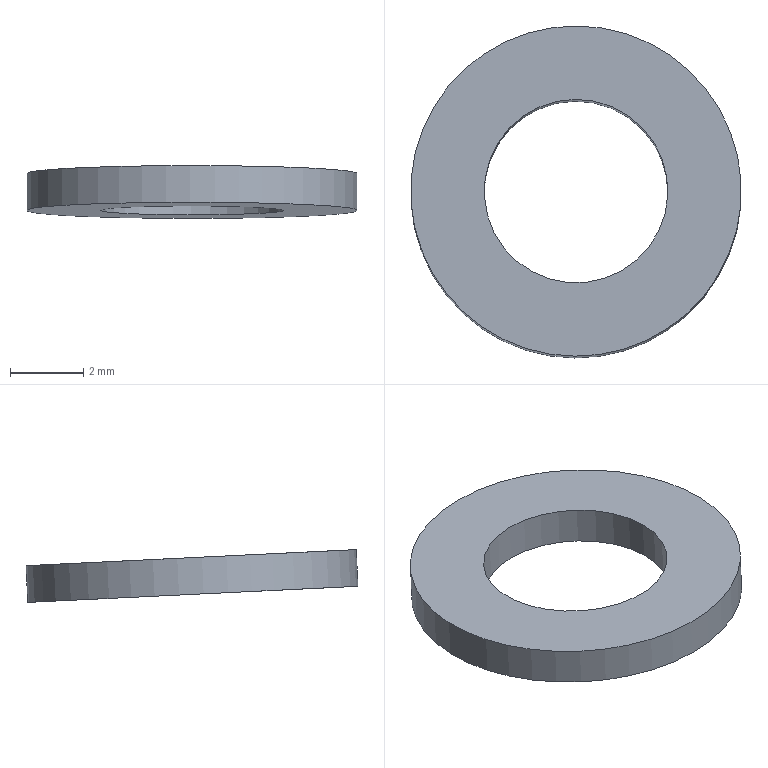Component | NX | CCJ-023 | 1 solid | 4 faces | box 9 x 9.04 x 1.44 mm | volume 44 mm3 | plane 2 | cylinder 2 | commonest cylinder face diameters 9 x1 5 x1
STEP:
#1=CARTESIAN_POINT('',(0.,0.,0.));
#2=DIRECTION('',(0.,0.,1.));
#3=DIRECTION('',(1.,0.,0.));
#4=AXIS2_PLACEMENT_3D('',#1,#2,#3);
#5=CARTESIAN_POINT('',(14.204,431.357,209.068));
#6=VERTEX_POINT('',#5);
#7=CARTESIAN_POINT('',(10.,429.754,209.146));
#8=DIRECTION('',(0.,-0.04861,-0.9988));
#9=DIRECTION('',(0.9342,0.3563,-0.01734));
#10=AXIS2_PLACEMENT_3D('',#7,#8,#9);
#11=CIRCLE('',#10,4.5);
#12=CARTESIAN_POINT('',(10.,429.754,209.146));
#13=DIRECTION('',(0.,0.04861,0.9988));
#14=DIRECTION('',(-0.9342,-0.3563,0.01734));
#15=AXIS2_PLACEMENT_3D('',#12,#13,#14);
#16=PLANE('',#15);
#17=CARTESIAN_POINT('',(-4.5,0.));
#18=CARTESIAN_POINT('',(-4.5,7.794));
#19=CARTESIAN_POINT('',(2.25,3.897));
#20=CARTESIAN_POINT('',(9.,-0.));
#21=CARTESIAN_POINT('',(2.25,-3.897));
#22=CARTESIAN_POINT('',(-4.5,-7.794));
#23=CARTESIAN_POINT('',(-4.5,0.));
#24=(BOUNDED_CURVE()B_SPLINE_CURVE(2,(#17,#18,#19,#20,#21,#22,#23),.UNSPECIFIED.,.T.,.F.)B_SPLINE_CURVE_WITH_KNOTS((1,2,2,2,2,1),(-2.094,0.,2.094,4.189,6.283,8.378),.UNSPECIFIED.)CURVE()GEOMETRIC_REPRESENTATION_ITEM()RATIONAL_B_SPLINE_CURVE((1.,0.5,1.,0.5,1.,0.5,1.))REPRESENTATION_ITEM(''));
#25=(GEOMETRIC_REPRESENTATION_CONTEXT(2)PARAMETRIC_REPRESENTATION_CONTEXT()REPRESENTATION_CONTEXT('',''));
#26=DEFINITIONAL_REPRESENTATION('',(#24),#25);
#27=PCURVE('',#16,#26);
#28=CARTESIAN_POINT('',(10.,429.754,209.146));
#29=DIRECTION('',(0.,-0.04861,-0.9988));
#30=DIRECTION('',(0.9342,0.3563,-0.01734));
#31=AXIS2_PLACEMENT_3D('',#28,#29,#30);
#32=CYLINDRICAL_SURFACE('',#31,4.5);
#33=CARTESIAN_POINT('',(0.,0.));
#34=DIRECTION('',(1.,0.));
#35=VECTOR('',#34,1.);
#36=LINE('',#33,#35);
#37=(GEOMETRIC_REPRESENTATION_CONTEXT(2)PARAMETRIC_REPRESENTATION_CONTEXT()REPRESENTATION_CONTEXT('',''));
#38=DEFINITIONAL_REPRESENTATION('',(#36),#37);
#39=PCURVE('',#32,#38);
#40=SURFACE_CURVE('',#11,(#27,#39),.PCURVE_S1.);
#41=EDGE_CURVE('',#6,#6,#40,.T.);
#42=ORIENTED_EDGE('',*,*,#41,.F.);
#43=EDGE_LOOP('',(#42));
#44=FACE_BOUND('',#43,.T.);
#45=CARTESIAN_POINT('',(12.336,430.645,209.103));
#46=VERTEX_POINT('',#45);
#47=CARTESIAN_POINT('',(10.,429.754,209.146));
#48=DIRECTION('',(0.,-0.04861,-0.9988));
#49=DIRECTION('',(0.9342,0.3563,-0.01734));
#50=AXIS2_PLACEMENT_3D('',#47,#48,#49);
#51=CIRCLE('',#50,2.5);
#52=CARTESIAN_POINT('',(-2.5,-0.));
#53=CARTESIAN_POINT('',(-2.5,4.33));
#54=CARTESIAN_POINT('',(1.25,2.165));
#55=CARTESIAN_POINT('',(5.,0.));
#56=CARTESIAN_POINT('',(1.25,-2.165));
#57=CARTESIAN_POINT('',(-2.5,-4.33));
#58=CARTESIAN_POINT('',(-2.5,-0.));
#59=(BOUNDED_CURVE()B_SPLINE_CURVE(2,(#52,#53,#54,#55,#56,#57,#58),.UNSPECIFIED.,.T.,.F.)B_SPLINE_CURVE_WITH_KNOTS((1,2,2,2,2,1),(-2.094,0.,2.094,4.189,6.283,8.378),.UNSPECIFIED.)CURVE()GEOMETRIC_REPRESENTATION_ITEM()RATIONAL_B_SPLINE_CURVE((1.,0.5,1.,0.5,1.,0.5,1.))REPRESENTATION_ITEM(''));
#60=(GEOMETRIC_REPRESENTATION_CONTEXT(2)PARAMETRIC_REPRESENTATION_CONTEXT()REPRESENTATION_CONTEXT('',''));
#61=DEFINITIONAL_REPRESENTATION('',(#59),#60);
#62=PCURVE('',#16,#61);
#63=CARTESIAN_POINT('',(10.,429.754,209.146));
#64=DIRECTION('',(0.,-0.04861,-0.9988));
#65=DIRECTION('',(0.9342,0.3563,-0.01734));
#66=AXIS2_PLACEMENT_3D('',#63,#64,#65);
#67=CYLINDRICAL_SURFACE('',#66,2.5);
#68=CARTESIAN_POINT('',(0.,-0.));
#69=DIRECTION('',(1.,0.));
#70=VECTOR('',#69,1.);
#71=LINE('',#68,#70);
#72=(GEOMETRIC_REPRESENTATION_CONTEXT(2)PARAMETRIC_REPRESENTATION_CONTEXT()REPRESENTATION_CONTEXT('',''));
#73=DEFINITIONAL_REPRESENTATION('',(#71),#72);
#74=PCURVE('',#67,#73);
#75=SURFACE_CURVE('',#51,(#62,#74),.PCURVE_S1.);
#76=EDGE_CURVE('',#46,#46,#75,.T.);
#77=ORIENTED_EDGE('',*,*,#76,.T.);
#78=EDGE_LOOP('',(#77));
#79=FACE_BOUND('',#78,.T.);
#80=ADVANCED_FACE('',(#44,#79),#16,.T.);
#81=CARTESIAN_POINT('',(14.204,431.309,208.069));
#82=VERTEX_POINT('',#81);
#83=CARTESIAN_POINT('',(10.,429.705,208.147));
#84=DIRECTION('',(0.,-0.04861,-0.9988));
#85=DIRECTION('',(0.9342,0.3563,-0.01734));
#86=AXIS2_PLACEMENT_3D('',#83,#84,#85);
#87=CIRCLE('',#86,4.5);
#88=CARTESIAN_POINT('',(10.,429.705,208.147));
#89=DIRECTION('',(0.,0.04861,0.9988));
#90=DIRECTION('',(-0.9342,-0.3563,0.01734));
#91=AXIS2_PLACEMENT_3D('',#88,#89,#90);
#92=PLANE('',#91);
#93=CARTESIAN_POINT('',(-4.5,0.));
#94=CARTESIAN_POINT('',(-4.5,7.794));
#95=CARTESIAN_POINT('',(2.25,3.897));
#96=CARTESIAN_POINT('',(9.,-0.));
#97=CARTESIAN_POINT('',(2.25,-3.897));
#98=CARTESIAN_POINT('',(-4.5,-7.794));
#99=CARTESIAN_POINT('',(-4.5,0.));
#100=(BOUNDED_CURVE()B_SPLINE_CURVE(2,(#93,#94,#95,#96,#97,#98,#99),.UNSPECIFIED.,.T.,.F.)B_SPLINE_CURVE_WITH_KNOTS((1,2,2,2,2,1),(-2.094,0.,2.094,4.189,6.283,8.378),.UNSPECIFIED.)CURVE()GEOMETRIC_REPRESENTATION_ITEM()RATIONAL_B_SPLINE_CURVE((1.,0.5,1.,0.5,1.,0.5,1.))REPRESENTATION_ITEM(''));
#101=(GEOMETRIC_REPRESENTATION_CONTEXT(2)PARAMETRIC_REPRESENTATION_CONTEXT()REPRESENTATION_CONTEXT('',''));
#102=DEFINITIONAL_REPRESENTATION('',(#100),#101);
#103=PCURVE('',#92,#102);
#104=CARTESIAN_POINT('',(0.,1.));
#105=DIRECTION('',(1.,0.));
#106=VECTOR('',#105,1.);
#107=LINE('',#104,#106);
#108=(GEOMETRIC_REPRESENTATION_CONTEXT(2)PARAMETRIC_REPRESENTATION_CONTEXT()REPRESENTATION_CONTEXT('',''));
#109=DEFINITIONAL_REPRESENTATION('',(#107),#108);
#110=PCURVE('',#32,#109);
#111=SURFACE_CURVE('',#87,(#103,#110),.PCURVE_S1.);
#112=EDGE_CURVE('',#82,#82,#111,.T.);
#113=ORIENTED_EDGE('',*,*,#112,.T.);
#114=EDGE_LOOP('',(#113));
#115=FACE_BOUND('',#114,.T.);
#116=CARTESIAN_POINT('',(12.336,430.596,208.104));
#117=VERTEX_POINT('',#116);
#118=CARTESIAN_POINT('',(10.,429.705,208.147));
#119=DIRECTION('',(0.,-0.04861,-0.9988));
#120=DIRECTION('',(0.9342,0.3563,-0.01734));
#121=AXIS2_PLACEMENT_3D('',#118,#119,#120);
#122=CIRCLE('',#121,2.5);
#123=CARTESIAN_POINT('',(-2.5,-0.));
#124=CARTESIAN_POINT('',(-2.5,4.33));
#125=CARTESIAN_POINT('',(1.25,2.165));
#126=CARTESIAN_POINT('',(5.,0.));
#127=CARTESIAN_POINT('',(1.25,-2.165));
#128=CARTESIAN_POINT('',(-2.5,-4.33));
#129=CARTESIAN_POINT('',(-2.5,-0.));
#130=(BOUNDED_CURVE()B_SPLINE_CURVE(2,(#123,#124,#125,#126,#127,#128,#129),.UNSPECIFIED.,.T.,.F.)B_SPLINE_CURVE_WITH_KNOTS((1,2,2,2,2,1),(-2.094,0.,2.094,4.189,6.283,8.378),.UNSPECIFIED.)CURVE()GEOMETRIC_REPRESENTATION_ITEM()RATIONAL_B_SPLINE_CURVE((1.,0.5,1.,0.5,1.,0.5,1.))REPRESENTATION_ITEM(''));
#131=(GEOMETRIC_REPRESENTATION_CONTEXT(2)PARAMETRIC_REPRESENTATION_CONTEXT()REPRESENTATION_CONTEXT('',''));
#132=DEFINITIONAL_REPRESENTATION('',(#130),#131);
#133=PCURVE('',#92,#132);
#134=CARTESIAN_POINT('',(0.,1.));
#135=DIRECTION('',(1.,0.));
#136=VECTOR('',#135,1.);
#137=LINE('',#134,#136);
#138=(GEOMETRIC_REPRESENTATION_CONTEXT(2)PARAMETRIC_REPRESENTATION_CONTEXT()REPRESENTATION_CONTEXT('',''));
#139=DEFINITIONAL_REPRESENTATION('',(#137),#138);
#140=PCURVE('',#67,#139);
#141=SURFACE_CURVE('',#122,(#133,#140),.PCURVE_S1.);
#142=EDGE_CURVE('',#117,#117,#141,.T.);
#143=ORIENTED_EDGE('',*,*,#142,.F.);
#144=EDGE_LOOP('',(#143));
#145=FACE_BOUND('',#144,.T.);
#146=ADVANCED_FACE('',(#115,#145),#92,.F.);
#147=ORIENTED_EDGE('',*,*,#41,.T.);
#148=CARTESIAN_POINT('',(14.204,431.357,209.068));
#149=CARTESIAN_POINT('',(14.204,431.309,208.069));
#150=B_SPLINE_CURVE_WITH_KNOTS('',1,(#148,#149),.UNSPECIFIED.,.F.,.F.,(2,2),(0.,1.),.PIECEWISE_BEZIER_KNOTS.);
#151=CARTESIAN_POINT('',(6.283,0.));
#152=DIRECTION('',(0.,1.));
#153=VECTOR('',#152,1.);
#154=LINE('',#151,#153);
#155=(GEOMETRIC_REPRESENTATION_CONTEXT(2)PARAMETRIC_REPRESENTATION_CONTEXT()REPRESENTATION_CONTEXT('',''));
#156=DEFINITIONAL_REPRESENTATION('',(#154),#155);
#157=PCURVE('',#32,#156);
#158=CARTESIAN_POINT('',(0.,0.));
#159=DIRECTION('',(0.,1.));
#160=VECTOR('',#159,1.);
#161=LINE('',#158,#160);
#162=(GEOMETRIC_REPRESENTATION_CONTEXT(2)PARAMETRIC_REPRESENTATION_CONTEXT()REPRESENTATION_CONTEXT('',''));
#163=DEFINITIONAL_REPRESENTATION('',(#161),#162);
#164=PCURVE('',#32,#163);
#165=SEAM_CURVE('',#150,(#157,#164),.PCURVE_S1.);
#166=EDGE_CURVE('',#6,#82,#165,.T.);
#167=ORIENTED_EDGE('',*,*,#166,.T.);
#168=ORIENTED_EDGE('',*,*,#112,.F.);
#169=ORIENTED_EDGE('',*,*,#166,.F.);
#170=EDGE_LOOP('',(#147,#167,#168,#169));
#171=FACE_BOUND('',#170,.T.);
#172=ADVANCED_FACE('',(#171),#32,.T.);
#173=ORIENTED_EDGE('',*,*,#76,.T.);
#174=CARTESIAN_POINT('',(12.336,430.645,209.103));
#175=CARTESIAN_POINT('',(12.336,430.596,208.104));
#176=B_SPLINE_CURVE_WITH_KNOTS('',1,(#174,#175),.UNSPECIFIED.,.F.,.F.,(2,2),(-0.,1.),.PIECEWISE_BEZIER_KNOTS.);
#177=CARTESIAN_POINT('',(6.283,0.));
#178=DIRECTION('',(0.,1.));
#179=VECTOR('',#178,1.);
#180=LINE('',#177,#179);
#181=(GEOMETRIC_REPRESENTATION_CONTEXT(2)PARAMETRIC_REPRESENTATION_CONTEXT()REPRESENTATION_CONTEXT('',''));
#182=DEFINITIONAL_REPRESENTATION('',(#180),#181);
#183=PCURVE('',#67,#182);
#184=CARTESIAN_POINT('',(0.,0.));
#185=DIRECTION('',(0.,1.));
#186=VECTOR('',#185,1.);
#187=LINE('',#184,#186);
#188=(GEOMETRIC_REPRESENTATION_CONTEXT(2)PARAMETRIC_REPRESENTATION_CONTEXT()REPRESENTATION_CONTEXT('',''));
#189=DEFINITIONAL_REPRESENTATION('',(#187),#188);
#190=PCURVE('',#67,#189);
#191=SEAM_CURVE('',#176,(#183,#190),.PCURVE_S1.);
#192=EDGE_CURVE('',#46,#117,#191,.T.);
#193=ORIENTED_EDGE('',*,*,#192,.T.);
#194=ORIENTED_EDGE('',*,*,#142,.F.);
#195=ORIENTED_EDGE('',*,*,#192,.F.);
#196=EDGE_LOOP('',(#173,#193,#194,#195));
#197=FACE_BOUND('',#196,.F.);
#198=ADVANCED_FACE('',(#197),#67,.F.);
#199=CLOSED_SHELL('',(#80,#146,#172,#198));
#200=MANIFOLD_SOLID_BREP('',#199);
#201=(LENGTH_UNIT()NAMED_UNIT(*)SI_UNIT(.MILLI.,.METRE.));
#202=UNCERTAINTY_MEASURE_WITH_UNIT(LENGTH_MEASURE(0.00001),#201,'','');
#203=(NAMED_UNIT(*)PLANE_ANGLE_UNIT()SI_UNIT($,.RADIAN.));
#204=(NAMED_UNIT(*)SI_UNIT($,.STERADIAN.)SOLID_ANGLE_UNIT());
#205=(GEOMETRIC_REPRESENTATION_CONTEXT(3)GLOBAL_UNCERTAINTY_ASSIGNED_CONTEXT((#202))GLOBAL_UNIT_ASSIGNED_CONTEXT((#201,#203,#204))REPRESENTATION_CONTEXT('',''));
#206=ADVANCED_BREP_SHAPE_REPRESENTATION('',(#4,#200),#205);